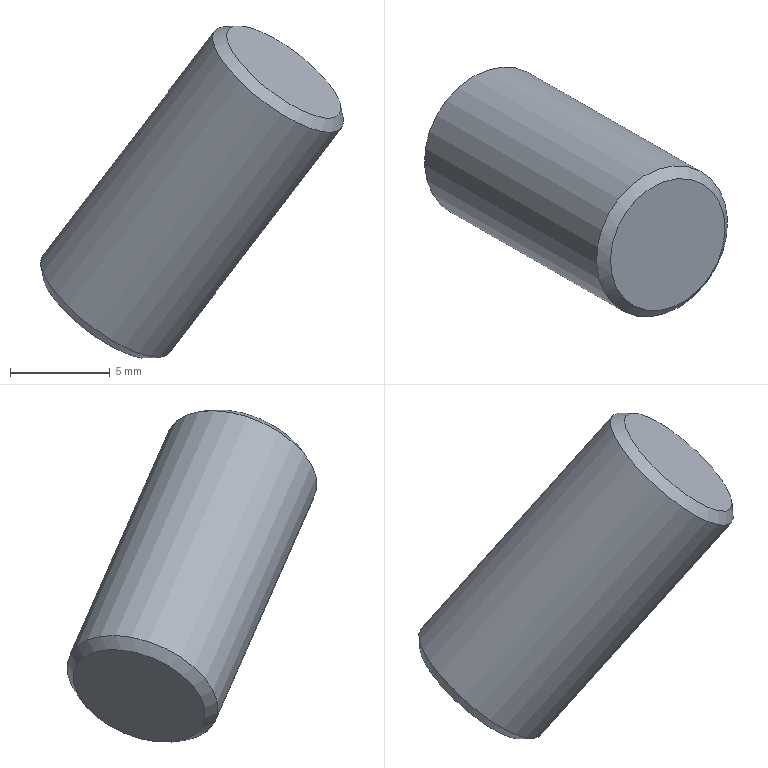Component | NX | XUANZHUAN_1 | 1 solid | 5 faces | box 15.16 x 12.5 x 16.63 mm | volume 798 mm3 | plane 2 | cone 2 | cylinder 1 | commonest cylinder face diameters 8 x1
STEP:
#1=CARTESIAN_POINT('',(0.,0.,0.));
#2=DIRECTION('',(0.,0.,1.));
#3=DIRECTION('',(1.,0.,0.));
#4=AXIS2_PLACEMENT_3D('',#1,#2,#3);
#5=CARTESIAN_POINT('',(-192.38,-42.202,79.259));
#6=VERTEX_POINT('',#5);
#7=CARTESIAN_POINT('',(-193.636,-45.938,78.574));
#8=DIRECTION('',(-0.5736,0.3301,-0.7497));
#9=DIRECTION('',(0.3138,0.9339,0.1711));
#10=AXIS2_PLACEMENT_3D('',#7,#8,#9);
#11=CIRCLE('',#10,4.);
#12=CARTESIAN_POINT('',(-202.526,-40.822,66.954));
#13=DIRECTION('',(0.5736,-0.3301,0.7497));
#14=DIRECTION('',(-0.3138,-0.9339,-0.1711));
#15=AXIS2_PLACEMENT_3D('',#12,#13,#14);
#16=CYLINDRICAL_SURFACE('',#15,4.);
#17=CARTESIAN_POINT('',(9.425,15.5));
#18=DIRECTION('',(-1.,0.));
#19=VECTOR('',#18,1.);
#20=LINE('',#17,#19);
#21=(GEOMETRIC_REPRESENTATION_CONTEXT(2)PARAMETRIC_REPRESENTATION_CONTEXT()REPRESENTATION_CONTEXT('',''));
#22=DEFINITIONAL_REPRESENTATION('',(#20),#21);
#23=PCURVE('',#16,#22);
#24=CARTESIAN_POINT('',(-193.636,-45.938,78.574));
#25=DIRECTION('',(-0.5736,0.3301,-0.7497));
#26=DIRECTION('',(0.3138,0.9339,0.1711));
#27=AXIS2_PLACEMENT_3D('',#24,#25,#26);
#28=CONICAL_SURFACE('',#27,4.,0.7854);
#29=CARTESIAN_POINT('',(0.,-0.));
#30=DIRECTION('',(1.,0.));
#31=VECTOR('',#30,1.);
#32=LINE('',#29,#31);
#33=(GEOMETRIC_REPRESENTATION_CONTEXT(2)PARAMETRIC_REPRESENTATION_CONTEXT()REPRESENTATION_CONTEXT('',''));
#34=DEFINITIONAL_REPRESENTATION('',(#32),#33);
#35=PCURVE('',#28,#34);
#36=SURFACE_CURVE('',#11,(#23,#35),.PCURVE_S1.);
#37=EDGE_CURVE('',#6,#6,#36,.T.);
#38=ORIENTED_EDGE('',*,*,#37,.T.);
#39=CARTESIAN_POINT('',(-200.984,-37.251,68.013));
#40=VERTEX_POINT('',#39);
#41=CARTESIAN_POINT('',(-200.984,-37.251,68.013));
#42=CARTESIAN_POINT('',(-192.38,-42.202,79.259));
#43=B_SPLINE_CURVE_WITH_KNOTS('',1,(#41,#42),.UNSPECIFIED.,.F.,.F.,(2,2),(0.5,15.5),.PIECEWISE_BEZIER_KNOTS.);
#44=CARTESIAN_POINT('',(3.142,0.));
#45=DIRECTION('',(0.,1.));
#46=VECTOR('',#45,1.);
#47=LINE('',#44,#46);
#48=(GEOMETRIC_REPRESENTATION_CONTEXT(2)PARAMETRIC_REPRESENTATION_CONTEXT()REPRESENTATION_CONTEXT('',''));
#49=DEFINITIONAL_REPRESENTATION('',(#47),#48);
#50=PCURVE('',#16,#49);
#51=CARTESIAN_POINT('',(9.425,0.));
#52=DIRECTION('',(0.,1.));
#53=VECTOR('',#52,1.);
#54=LINE('',#51,#53);
#55=(GEOMETRIC_REPRESENTATION_CONTEXT(2)PARAMETRIC_REPRESENTATION_CONTEXT()REPRESENTATION_CONTEXT('',''));
#56=DEFINITIONAL_REPRESENTATION('',(#54),#55);
#57=PCURVE('',#16,#56);
#58=SEAM_CURVE('',#43,(#50,#57),.PCURVE_S1.);
#59=EDGE_CURVE('',#40,#6,#58,.T.);
#60=ORIENTED_EDGE('',*,*,#59,.F.);
#61=CARTESIAN_POINT('',(-202.239,-40.987,67.328));
#62=DIRECTION('',(0.5736,-0.3301,0.7497));
#63=DIRECTION('',(0.3138,0.9339,0.1711));
#64=AXIS2_PLACEMENT_3D('',#61,#62,#63);
#65=CIRCLE('',#64,4.);
#66=CARTESIAN_POINT('',(3.142,0.5));
#67=DIRECTION('',(1.,0.));
#68=VECTOR('',#67,1.);
#69=LINE('',#66,#68);
#70=(GEOMETRIC_REPRESENTATION_CONTEXT(2)PARAMETRIC_REPRESENTATION_CONTEXT()REPRESENTATION_CONTEXT('',''));
#71=DEFINITIONAL_REPRESENTATION('',(#69),#70);
#72=PCURVE('',#16,#71);
#73=CARTESIAN_POINT('',(-202.526,-40.822,66.954));
#74=DIRECTION('',(0.5736,-0.3301,0.7497));
#75=DIRECTION('',(-0.3138,-0.9339,-0.1711));
#76=AXIS2_PLACEMENT_3D('',#73,#74,#75);
#77=CONICAL_SURFACE('',#76,3.5,0.7854);
#78=CARTESIAN_POINT('',(3.142,0.5));
#79=DIRECTION('',(1.,0.));
#80=VECTOR('',#79,1.);
#81=LINE('',#78,#80);
#82=(GEOMETRIC_REPRESENTATION_CONTEXT(2)PARAMETRIC_REPRESENTATION_CONTEXT()REPRESENTATION_CONTEXT('',''));
#83=DEFINITIONAL_REPRESENTATION('',(#81),#82);
#84=PCURVE('',#77,#83);
#85=SURFACE_CURVE('',#65,(#72,#84),.PCURVE_S1.);
#86=EDGE_CURVE('',#40,#40,#85,.T.);
#87=ORIENTED_EDGE('',*,*,#86,.T.);
#88=ORIENTED_EDGE('',*,*,#59,.T.);
#89=EDGE_LOOP('',(#38,#60,#87,#88));
#90=FACE_BOUND('',#89,.T.);
#91=ADVANCED_FACE('',(#90),#16,.T.);
#92=CARTESIAN_POINT('',(-201.428,-37.553,67.552));
#93=VERTEX_POINT('',#92);
#94=CARTESIAN_POINT('',(-202.526,-40.822,66.954));
#95=DIRECTION('',(-0.5736,0.3301,-0.7497));
#96=DIRECTION('',(0.3138,0.9339,0.1711));
#97=AXIS2_PLACEMENT_3D('',#94,#95,#96);
#98=CIRCLE('',#97,3.5);
#99=CARTESIAN_POINT('',(-202.526,-40.822,66.954));
#100=DIRECTION('',(-0.5736,0.3301,-0.7497));
#101=DIRECTION('',(0.3138,0.9339,0.1711));
#102=AXIS2_PLACEMENT_3D('',#99,#100,#101);
#103=PLANE('',#102);
#104=CARTESIAN_POINT('',(0.,0.));
#105=DIRECTION('',(1.,-0.));
#106=AXIS2_PLACEMENT_2D('',#104,#105);
#107=CIRCLE('',#106,3.5);
#108=(GEOMETRIC_REPRESENTATION_CONTEXT(2)PARAMETRIC_REPRESENTATION_CONTEXT()REPRESENTATION_CONTEXT('',''));
#109=DEFINITIONAL_REPRESENTATION('',(#107),#108);
#110=PCURVE('',#103,#109);
#111=CARTESIAN_POINT('',(9.425,-0.));
#112=DIRECTION('',(-1.,0.));
#113=VECTOR('',#112,1.);
#114=LINE('',#111,#113);
#115=(GEOMETRIC_REPRESENTATION_CONTEXT(2)PARAMETRIC_REPRESENTATION_CONTEXT()REPRESENTATION_CONTEXT('',''));
#116=DEFINITIONAL_REPRESENTATION('',(#114),#115);
#117=PCURVE('',#77,#116);
#118=SURFACE_CURVE('',#98,(#110,#117),.PCURVE_S1.);
#119=EDGE_CURVE('',#93,#93,#118,.T.);
#120=ORIENTED_EDGE('',*,*,#119,.T.);
#121=EDGE_LOOP('',(#120));
#122=FACE_BOUND('',#121,.T.);
#123=ADVANCED_FACE('',(#122),#103,.T.);
#124=CARTESIAN_POINT('',(-192.251,-42.834,79.548));
#125=VERTEX_POINT('',#124);
#126=CARTESIAN_POINT('',(-193.349,-46.103,78.949));
#127=DIRECTION('',(0.5736,-0.3301,0.7497));
#128=DIRECTION('',(0.3138,0.9339,0.1711));
#129=AXIS2_PLACEMENT_3D('',#126,#127,#128);
#130=CIRCLE('',#129,3.5);
#131=CARTESIAN_POINT('',(-193.349,-46.103,78.949));
#132=DIRECTION('',(-0.5736,0.3301,-0.7497));
#133=DIRECTION('',(0.3138,0.9339,0.1711));
#134=AXIS2_PLACEMENT_3D('',#131,#132,#133);
#135=PLANE('',#134);
#136=CARTESIAN_POINT('',(3.5,-0.));
#137=CARTESIAN_POINT('',(3.5,-6.062));
#138=CARTESIAN_POINT('',(-1.75,-3.031));
#139=CARTESIAN_POINT('',(-7.,0.));
#140=CARTESIAN_POINT('',(-1.75,3.031));
#141=CARTESIAN_POINT('',(3.5,6.062));
#142=CARTESIAN_POINT('',(3.5,-0.));
#143=(BOUNDED_CURVE()B_SPLINE_CURVE(2,(#136,#137,#138,#139,#140,#141,#142),.UNSPECIFIED.,.T.,.F.)B_SPLINE_CURVE_WITH_KNOTS((1,2,2,2,2,1),(-2.094,0.,2.094,4.189,6.283,8.378),.UNSPECIFIED.)CURVE()GEOMETRIC_REPRESENTATION_ITEM()RATIONAL_B_SPLINE_CURVE((1.,0.5,1.,0.5,1.,0.5,1.))REPRESENTATION_ITEM(''));
#144=(GEOMETRIC_REPRESENTATION_CONTEXT(2)PARAMETRIC_REPRESENTATION_CONTEXT()REPRESENTATION_CONTEXT('',''));
#145=DEFINITIONAL_REPRESENTATION('',(#143),#144);
#146=PCURVE('',#135,#145);
#147=CARTESIAN_POINT('',(6.283,-0.5));
#148=DIRECTION('',(-1.,0.));
#149=VECTOR('',#148,1.);
#150=LINE('',#147,#149);
#151=(GEOMETRIC_REPRESENTATION_CONTEXT(2)PARAMETRIC_REPRESENTATION_CONTEXT()REPRESENTATION_CONTEXT('',''));
#152=DEFINITIONAL_REPRESENTATION('',(#150),#151);
#153=PCURVE('',#28,#152);
#154=SURFACE_CURVE('',#130,(#146,#153),.PCURVE_S1.);
#155=EDGE_CURVE('',#125,#125,#154,.T.);
#156=ORIENTED_EDGE('',*,*,#155,.T.);
#157=EDGE_LOOP('',(#156));
#158=FACE_BOUND('',#157,.T.);
#159=ADVANCED_FACE('',(#158),#135,.F.);
#160=ORIENTED_EDGE('',*,*,#86,.F.);
#161=CARTESIAN_POINT('',(-201.428,-37.553,67.552));
#162=CARTESIAN_POINT('',(-200.984,-37.251,68.013));
#163=B_SPLINE_CURVE_WITH_KNOTS('',1,(#161,#162),.UNSPECIFIED.,.F.,.F.,(2,2),(-0.,0.7071),.PIECEWISE_BEZIER_KNOTS.);
#164=CARTESIAN_POINT('',(3.142,0.));
#165=DIRECTION('',(0.,1.));
#166=VECTOR('',#165,1.);
#167=LINE('',#164,#166);
#168=(GEOMETRIC_REPRESENTATION_CONTEXT(2)PARAMETRIC_REPRESENTATION_CONTEXT()REPRESENTATION_CONTEXT('',''));
#169=DEFINITIONAL_REPRESENTATION('',(#167),#168);
#170=PCURVE('',#77,#169);
#171=CARTESIAN_POINT('',(9.425,0.));
#172=DIRECTION('',(0.,1.));
#173=VECTOR('',#172,1.);
#174=LINE('',#171,#173);
#175=(GEOMETRIC_REPRESENTATION_CONTEXT(2)PARAMETRIC_REPRESENTATION_CONTEXT()REPRESENTATION_CONTEXT('',''));
#176=DEFINITIONAL_REPRESENTATION('',(#174),#175);
#177=PCURVE('',#77,#176);
#178=SEAM_CURVE('',#163,(#170,#177),.PCURVE_S1.);
#179=EDGE_CURVE('',#93,#40,#178,.T.);
#180=ORIENTED_EDGE('',*,*,#179,.F.);
#181=ORIENTED_EDGE('',*,*,#119,.F.);
#182=ORIENTED_EDGE('',*,*,#179,.T.);
#183=EDGE_LOOP('',(#160,#180,#181,#182));
#184=FACE_BOUND('',#183,.T.);
#185=ADVANCED_FACE('',(#184),#77,.T.);
#186=ORIENTED_EDGE('',*,*,#155,.F.);
#187=CARTESIAN_POINT('',(-192.251,-42.834,79.548));
#188=CARTESIAN_POINT('',(-192.38,-42.202,79.259));
#189=B_SPLINE_CURVE_WITH_KNOTS('',1,(#187,#188),.UNSPECIFIED.,.F.,.F.,(2,2),(-0.7071,-0.),.PIECEWISE_BEZIER_KNOTS.);
#190=CARTESIAN_POINT('',(6.283,0.));
#191=DIRECTION('',(0.,1.));
#192=VECTOR('',#191,1.);
#193=LINE('',#190,#192);
#194=(GEOMETRIC_REPRESENTATION_CONTEXT(2)PARAMETRIC_REPRESENTATION_CONTEXT()REPRESENTATION_CONTEXT('',''));
#195=DEFINITIONAL_REPRESENTATION('',(#193),#194);
#196=PCURVE('',#28,#195);
#197=CARTESIAN_POINT('',(0.,0.));
#198=DIRECTION('',(0.,1.));
#199=VECTOR('',#198,1.);
#200=LINE('',#197,#199);
#201=(GEOMETRIC_REPRESENTATION_CONTEXT(2)PARAMETRIC_REPRESENTATION_CONTEXT()REPRESENTATION_CONTEXT('',''));
#202=DEFINITIONAL_REPRESENTATION('',(#200),#201);
#203=PCURVE('',#28,#202);
#204=SEAM_CURVE('',#189,(#196,#203),.PCURVE_S1.);
#205=EDGE_CURVE('',#125,#6,#204,.T.);
#206=ORIENTED_EDGE('',*,*,#205,.T.);
#207=ORIENTED_EDGE('',*,*,#37,.F.);
#208=ORIENTED_EDGE('',*,*,#205,.F.);
#209=EDGE_LOOP('',(#186,#206,#207,#208));
#210=FACE_BOUND('',#209,.T.);
#211=ADVANCED_FACE('',(#210),#28,.T.);
#212=CLOSED_SHELL('',(#91,#123,#159,#185,#211));
#213=MANIFOLD_SOLID_BREP('',#212);
#214=(LENGTH_UNIT()NAMED_UNIT(*)SI_UNIT(.MILLI.,.METRE.));
#215=UNCERTAINTY_MEASURE_WITH_UNIT(LENGTH_MEASURE(0.00001),#214,'','');
#216=(NAMED_UNIT(*)PLANE_ANGLE_UNIT()SI_UNIT($,.RADIAN.));
#217=(NAMED_UNIT(*)SI_UNIT($,.STERADIAN.)SOLID_ANGLE_UNIT());
#218=(GEOMETRIC_REPRESENTATION_CONTEXT(3)GLOBAL_UNCERTAINTY_ASSIGNED_CONTEXT((#215))GLOBAL_UNIT_ASSIGNED_CONTEXT((#214,#216,#217))REPRESENTATION_CONTEXT('',''));
#219=ADVANCED_BREP_SHAPE_REPRESENTATION('',(#4,#213),#218);